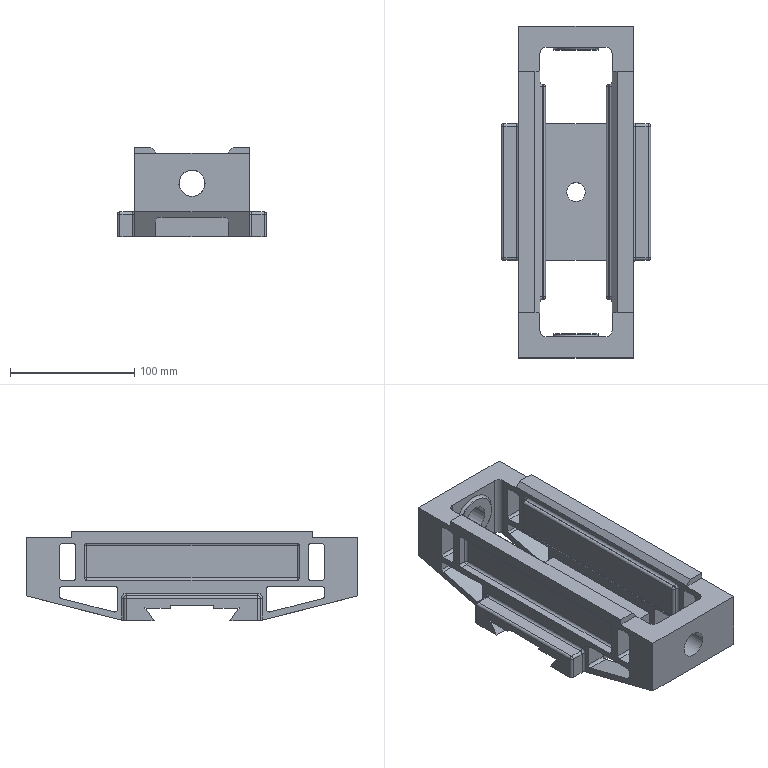Component | NX | MOVINGTABLE | 1 solid | 231 faces | volume 660962 mm3 | plane 100 | cylinder 97 | sphere 20 | torus 14 | commonest cylinder face diameters 4 x88 10 x4 21 x2 36 x2 15 x1